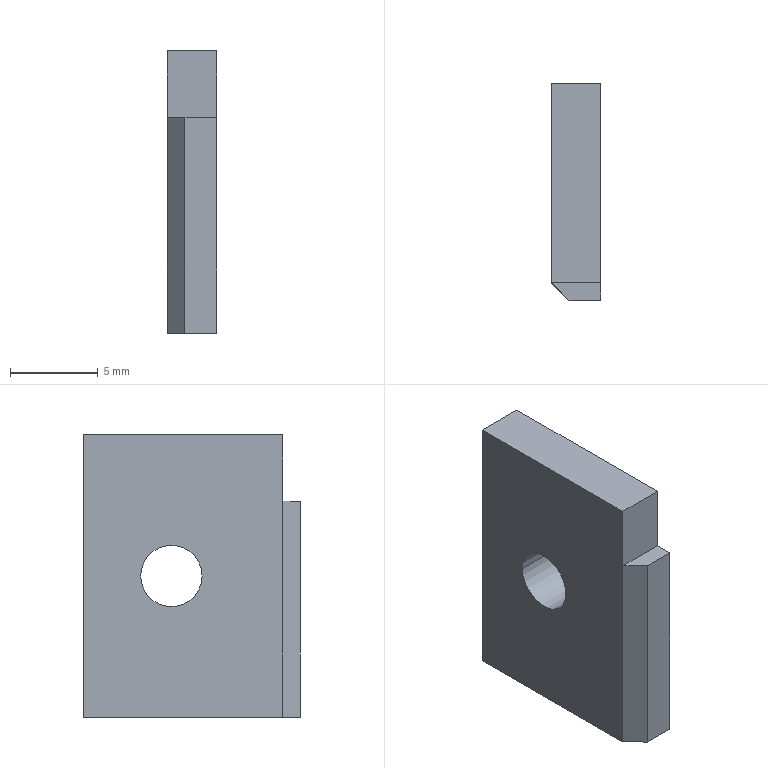Component | SolidWorks | 7.1.02.0001.00.00-0084-1 | 1 solid | 11 faces | box 2.8 x 12.35 x 16.1 mm | volume 513 mm3 | plane 9 | cylinder 2 | commonest cylinder face diameters 3.5 x2
build123d program:
from build123d import *

# Parameters (mm, degrees)
SKETCH1_W           = 12.35
SKETCH1_H           = 16.1
SKETCH1_R           = 1.75
BOSS_EXTRUDE1_DEPTH = 2.8
CHAMFER1_SIZE       = 1
SKETCH2_W           = 1
SKETCH2_H           = 3.8
CUT_EXTRUDE1_DEPTH  = 11.525


with BuildPart() as part:
    # Sketch1 → Boss-Extrude1 (new body)
    with BuildSketch(Plane.XY):
        Rectangle(SKETCH1_W, SKETCH1_H)
        with Locations((-1.175, 0)):
            Circle(SKETCH1_R, mode=Mode.SUBTRACT)
    extrude(amount=BOSS_EXTRUDE1_DEPTH)

    # Chamfer1
    chamfer1_edges = [part.edges().sort_by_distance(p)[0] for p in [
        (6.175, 0, 0),
    ]]
    chamfer(chamfer1_edges, length=CHAMFER1_SIZE)

    # Sketch2 → Cut-Extrude1 (cut, through all)
    with BuildSketch(Plane(origin=(0, 0, 0), x_dir=(-1, 0, 0), z_dir=(0, 0, -1))):
        with Locations((-5.675, -6.15)):
            Rectangle(SKETCH2_W, SKETCH2_H)
    extrude(amount=-CUT_EXTRUDE1_DEPTH, mode=Mode.SUBTRACT)


solid = part.part

# Placed as in the assembly
solid = solid.moved(Location((-67.964, 37.141, 0), (-90, 90, 0)))
STEP:
#1=COLOUR_RGB('',0.7922,0.8196,0.9333);
#2=FILL_AREA_STYLE_COLOUR('',#1);
#3=FILL_AREA_STYLE('',(#2));
#4=SURFACE_STYLE_FILL_AREA(#3);
#5=SURFACE_SIDE_STYLE('',(#4));
#6=SURFACE_STYLE_USAGE(.BOTH.,#5);
#7=PRESENTATION_STYLE_ASSIGNMENT((#6));
#8=CARTESIAN_POINT('',(-2.566,1.577,-0.));
#9=VERTEX_POINT('',#8);
#10=CARTESIAN_POINT('',(-2.566,1.44,-0.));
#11=VERTEX_POINT('',#10);
#12=CARTESIAN_POINT('',(-2.566,1.509,-0.));
#13=DIRECTION('',(1.,-0.,-0.));
#14=DIRECTION('',(0.,-1.,-0.));
#15=AXIS2_PLACEMENT_3D('',#12,#13,#14);
#16=CIRCLE('',#15,0.0689);
#17=EDGE_CURVE('',#9,#11,#16,.T.);
#18=ORIENTED_EDGE('',*,*,#17,.T.);
#19=CARTESIAN_POINT('',(-2.676,1.44,-0.));
#20=VERTEX_POINT('',#19);
#21=CARTESIAN_POINT('',(-2.566,1.44,-0.));
#22=DIRECTION('',(-1.,0.,0.));
#23=VECTOR('',#22,39.37);
#24=LINE('',#21,#23);
#25=EDGE_CURVE('',#11,#20,#24,.T.);
#26=ORIENTED_EDGE('',*,*,#25,.T.);
#27=CARTESIAN_POINT('',(-2.676,1.577,-0.));
#28=VERTEX_POINT('',#27);
#29=CARTESIAN_POINT('',(-2.676,1.509,-0.));
#30=DIRECTION('',(1.,-0.,-0.));
#31=DIRECTION('',(0.,-1.,-0.));
#32=AXIS2_PLACEMENT_3D('',#29,#30,#31);
#33=CIRCLE('',#32,0.0689);
#34=EDGE_CURVE('',#28,#20,#33,.T.);
#35=ORIENTED_EDGE('',*,*,#34,.F.);
#36=CARTESIAN_POINT('',(-2.566,1.577,-0.));
#37=DIRECTION('',(-1.,0.,0.));
#38=VECTOR('',#37,39.37);
#39=LINE('',#36,#38);
#40=EDGE_CURVE('',#9,#28,#39,.T.);
#41=ORIENTED_EDGE('',*,*,#40,.F.);
#42=EDGE_LOOP('',(#18,#26,#35,#41));
#43=FACE_OUTER_BOUND('',#42,.T.);
#44=CARTESIAN_POINT('',(-2.566,1.509,-0.));
#45=DIRECTION('',(-1.,0.,0.));
#46=DIRECTION('',(0.,1.,0.));
#47=AXIS2_PLACEMENT_3D('',#44,#45,#46);
#48=CYLINDRICAL_SURFACE('',#47,0.0689);
#49=ADVANCED_FACE('',(#43),#48,.F.);
#50=CARTESIAN_POINT('',(-2.566,1.259,0.1673));
#51=VERTEX_POINT('',#50);
#52=CARTESIAN_POINT('',(-2.566,1.219,0.1673));
#53=VERTEX_POINT('',#52);
#54=CARTESIAN_POINT('',(-2.566,1.219,0.1673));
#55=DIRECTION('',(-0.,-1.,-0.));
#56=VECTOR('',#55,39.37);
#57=LINE('',#54,#56);
#58=EDGE_CURVE('',#51,#53,#57,.T.);
#59=ORIENTED_EDGE('',*,*,#58,.T.);
#60=CARTESIAN_POINT('',(-2.566,1.219,-0.3169));
#61=VERTEX_POINT('',#60);
#62=CARTESIAN_POINT('',(-2.566,1.219,-0.3169));
#63=DIRECTION('',(-0.,0.,-1.));
#64=VECTOR('',#63,39.37);
#65=LINE('',#62,#64);
#66=EDGE_CURVE('',#53,#61,#65,.T.);
#67=ORIENTED_EDGE('',*,*,#66,.T.);
#68=CARTESIAN_POINT('',(-2.566,1.705,-0.3169));
#69=VERTEX_POINT('',#68);
#70=CARTESIAN_POINT('',(-2.566,1.705,-0.3169));
#71=DIRECTION('',(0.,1.,0.));
#72=VECTOR('',#71,39.37);
#73=LINE('',#70,#72);
#74=EDGE_CURVE('',#61,#69,#73,.T.);
#75=ORIENTED_EDGE('',*,*,#74,.T.);
#76=CARTESIAN_POINT('',(-2.566,1.705,0.3169));
#77=VERTEX_POINT('',#76);
#78=CARTESIAN_POINT('',(-2.566,1.705,-0.3169));
#79=DIRECTION('',(0.,-0.,1.));
#80=VECTOR('',#79,39.37);
#81=LINE('',#78,#80);
#82=EDGE_CURVE('',#69,#77,#81,.T.);
#83=ORIENTED_EDGE('',*,*,#82,.T.);
#84=CARTESIAN_POINT('',(-2.566,1.259,0.3169));
#85=VERTEX_POINT('',#84);
#86=CARTESIAN_POINT('',(-2.566,1.705,0.3169));
#87=DIRECTION('',(-0.,-1.,-0.));
#88=VECTOR('',#87,39.37);
#89=LINE('',#86,#88);
#90=EDGE_CURVE('',#77,#85,#89,.T.);
#91=ORIENTED_EDGE('',*,*,#90,.T.);
#92=CARTESIAN_POINT('',(-2.566,1.259,0.3169));
#93=DIRECTION('',(-0.,-0.,-1.));
#94=VECTOR('',#93,39.37);
#95=LINE('',#92,#94);
#96=EDGE_CURVE('',#85,#51,#95,.T.);
#97=ORIENTED_EDGE('',*,*,#96,.T.);
#98=EDGE_LOOP('',(#59,#67,#75,#83,#91,#97));
#99=FACE_OUTER_BOUND('',#98,.T.);
#100=ORIENTED_EDGE('',*,*,#17,.F.);
#101=CARTESIAN_POINT('',(-2.566,1.509,-0.));
#102=DIRECTION('',(1.,-0.,-0.));
#103=DIRECTION('',(0.,-1.,-0.));
#104=AXIS2_PLACEMENT_3D('',#101,#102,#103);
#105=CIRCLE('',#104,0.0689);
#106=EDGE_CURVE('',#11,#9,#105,.T.);
#107=ORIENTED_EDGE('',*,*,#106,.F.);
#108=EDGE_LOOP('',(#100,#107));
#109=FACE_BOUND('',#108,.T.);
#110=CARTESIAN_POINT('',(-2.566,1.462,-0.));
#111=DIRECTION('',(1.,-0.,-0.));
#112=DIRECTION('',(-0.,-1.,-0.));
#113=AXIS2_PLACEMENT_3D('',#110,#111,#112);
#114=PLANE('',#113);
#115=ADVANCED_FACE('',(#99,#109),#114,.T.);
#116=CARTESIAN_POINT('',(-2.676,1.259,-0.3169));
#117=VERTEX_POINT('',#116);
#118=CARTESIAN_POINT('',(-2.676,1.705,-0.3169));
#119=VERTEX_POINT('',#118);
#120=CARTESIAN_POINT('',(-2.676,1.705,-0.3169));
#121=DIRECTION('',(0.,1.,0.));
#122=VECTOR('',#121,39.37);
#123=LINE('',#120,#122);
#124=EDGE_CURVE('',#117,#119,#123,.T.);
#125=ORIENTED_EDGE('',*,*,#124,.F.);
#126=CARTESIAN_POINT('',(-2.676,1.259,0.1673));
#127=VERTEX_POINT('',#126);
#128=CARTESIAN_POINT('',(-2.676,1.259,-0.));
#129=DIRECTION('',(0.,-0.,1.));
#130=VECTOR('',#129,39.37);
#131=LINE('',#128,#130);
#132=EDGE_CURVE('',#117,#127,#131,.T.);
#133=ORIENTED_EDGE('',*,*,#132,.T.);
#134=CARTESIAN_POINT('',(-2.676,1.259,0.3169));
#135=VERTEX_POINT('',#134);
#136=CARTESIAN_POINT('',(-2.676,1.259,0.3169));
#137=DIRECTION('',(-0.,-0.,-1.));
#138=VECTOR('',#137,39.37);
#139=LINE('',#136,#138);
#140=EDGE_CURVE('',#135,#127,#139,.T.);
#141=ORIENTED_EDGE('',*,*,#140,.F.);
#142=CARTESIAN_POINT('',(-2.676,1.705,0.3169));
#143=VERTEX_POINT('',#142);
#144=CARTESIAN_POINT('',(-2.676,1.705,0.3169));
#145=DIRECTION('',(-0.,-1.,-0.));
#146=VECTOR('',#145,39.37);
#147=LINE('',#144,#146);
#148=EDGE_CURVE('',#143,#135,#147,.T.);
#149=ORIENTED_EDGE('',*,*,#148,.F.);
#150=CARTESIAN_POINT('',(-2.676,1.705,-0.3169));
#151=DIRECTION('',(0.,-0.,1.));
#152=VECTOR('',#151,39.37);
#153=LINE('',#150,#152);
#154=EDGE_CURVE('',#119,#143,#153,.T.);
#155=ORIENTED_EDGE('',*,*,#154,.F.);
#156=EDGE_LOOP('',(#125,#133,#141,#149,#155));
#157=FACE_OUTER_BOUND('',#156,.T.);
#158=ORIENTED_EDGE('',*,*,#34,.T.);
#159=CARTESIAN_POINT('',(-2.676,1.509,-0.));
#160=DIRECTION('',(1.,-0.,-0.));
#161=DIRECTION('',(0.,-1.,-0.));
#162=AXIS2_PLACEMENT_3D('',#159,#160,#161);
#163=CIRCLE('',#162,0.0689);
#164=EDGE_CURVE('',#20,#28,#163,.T.);
#165=ORIENTED_EDGE('',*,*,#164,.T.);
#166=EDGE_LOOP('',(#158,#165));
#167=FACE_BOUND('',#166,.T.);
#168=CARTESIAN_POINT('',(-2.676,1.462,-0.));
#169=DIRECTION('',(1.,-0.,-0.));
#170=DIRECTION('',(-0.,-1.,-0.));
#171=AXIS2_PLACEMENT_3D('',#168,#169,#170);
#172=PLANE('',#171);
#173=ADVANCED_FACE('',(#157,#167),#172,.F.);
#174=ORIENTED_EDGE('',*,*,#154,.T.);
#175=CARTESIAN_POINT('',(-2.566,1.705,0.3169));
#176=DIRECTION('',(-1.,0.,0.));
#177=VECTOR('',#176,39.37);
#178=LINE('',#175,#177);
#179=EDGE_CURVE('',#77,#143,#178,.T.);
#180=ORIENTED_EDGE('',*,*,#179,.F.);
#181=ORIENTED_EDGE('',*,*,#82,.F.);
#182=CARTESIAN_POINT('',(-2.566,1.705,-0.3169));
#183=DIRECTION('',(-1.,0.,0.));
#184=VECTOR('',#183,39.37);
#185=LINE('',#182,#184);
#186=EDGE_CURVE('',#69,#119,#185,.T.);
#187=ORIENTED_EDGE('',*,*,#186,.T.);
#188=EDGE_LOOP('',(#174,#180,#181,#187));
#189=FACE_OUTER_BOUND('',#188,.T.);
#190=CARTESIAN_POINT('',(-2.566,1.705,-0.3169));
#191=DIRECTION('',(-0.,-1.,-0.));
#192=DIRECTION('',(-1.,0.,0.));
#193=AXIS2_PLACEMENT_3D('',#190,#191,#192);
#194=PLANE('',#193);
#195=ADVANCED_FACE('',(#189),#194,.F.);
#196=ORIENTED_EDGE('',*,*,#148,.T.);
#197=CARTESIAN_POINT('',(-2.566,1.259,0.3169));
#198=DIRECTION('',(-1.,0.,0.));
#199=VECTOR('',#198,39.37);
#200=LINE('',#197,#199);
#201=EDGE_CURVE('',#85,#135,#200,.T.);
#202=ORIENTED_EDGE('',*,*,#201,.F.);
#203=ORIENTED_EDGE('',*,*,#90,.F.);
#204=ORIENTED_EDGE('',*,*,#179,.T.);
#205=EDGE_LOOP('',(#196,#202,#203,#204));
#206=FACE_OUTER_BOUND('',#205,.T.);
#207=CARTESIAN_POINT('',(-2.566,1.705,0.3169));
#208=DIRECTION('',(-0.,0.,-1.));
#209=DIRECTION('',(1.,-0.,-0.));
#210=AXIS2_PLACEMENT_3D('',#207,#208,#209);
#211=PLANE('',#210);
#212=ADVANCED_FACE('',(#206),#211,.F.);
#213=ORIENTED_EDGE('',*,*,#66,.F.);
#214=CARTESIAN_POINT('',(-2.636,1.219,0.1673));
#215=VERTEX_POINT('',#214);
#216=CARTESIAN_POINT('',(-2.566,1.219,0.1673));
#217=DIRECTION('',(-1.,0.,0.));
#218=VECTOR('',#217,39.37);
#219=LINE('',#216,#218);
#220=EDGE_CURVE('',#53,#215,#219,.T.);
#221=ORIENTED_EDGE('',*,*,#220,.T.);
#222=CARTESIAN_POINT('',(-2.636,1.219,-0.3169));
#223=VERTEX_POINT('',#222);
#224=CARTESIAN_POINT('',(-2.636,1.219,-0.3169));
#225=DIRECTION('',(-0.,0.,-1.));
#226=VECTOR('',#225,39.37);
#227=LINE('',#224,#226);
#228=EDGE_CURVE('',#215,#223,#227,.T.);
#229=ORIENTED_EDGE('',*,*,#228,.T.);
#230=CARTESIAN_POINT('',(-2.566,1.219,-0.3169));
#231=DIRECTION('',(-1.,0.,0.));
#232=VECTOR('',#231,39.37);
#233=LINE('',#230,#232);
#234=EDGE_CURVE('',#61,#223,#233,.T.);
#235=ORIENTED_EDGE('',*,*,#234,.F.);
#236=EDGE_LOOP('',(#213,#221,#229,#235));
#237=FACE_OUTER_BOUND('',#236,.T.);
#238=CARTESIAN_POINT('',(-2.566,1.219,-0.3169));
#239=DIRECTION('',(0.,1.,0.));
#240=DIRECTION('',(1.,-0.,-0.));
#241=AXIS2_PLACEMENT_3D('',#238,#239,#240);
#242=PLANE('',#241);
#243=ADVANCED_FACE('',(#237),#242,.F.);
#244=ORIENTED_EDGE('',*,*,#234,.T.);
#245=CARTESIAN_POINT('',(-2.636,1.219,-0.3169));
#246=DIRECTION('',(-0.7071,0.7071,0.));
#247=VECTOR('',#246,39.37);
#248=LINE('',#245,#247);
#249=EDGE_CURVE('',#223,#117,#248,.T.);
#250=ORIENTED_EDGE('',*,*,#249,.T.);
#251=ORIENTED_EDGE('',*,*,#124,.T.);
#252=ORIENTED_EDGE('',*,*,#186,.F.);
#253=ORIENTED_EDGE('',*,*,#74,.F.);
#254=EDGE_LOOP('',(#244,#250,#251,#252,#253));
#255=FACE_OUTER_BOUND('',#254,.T.);
#256=CARTESIAN_POINT('',(-2.566,1.705,-0.3169));
#257=DIRECTION('',(0.,-0.,1.));
#258=DIRECTION('',(-1.,0.,0.));
#259=AXIS2_PLACEMENT_3D('',#256,#257,#258);
#260=PLANE('',#259);
#261=ADVANCED_FACE('',(#255),#260,.F.);
#262=ORIENTED_EDGE('',*,*,#25,.F.);
#263=ORIENTED_EDGE('',*,*,#106,.T.);
#264=ORIENTED_EDGE('',*,*,#40,.T.);
#265=ORIENTED_EDGE('',*,*,#164,.F.);
#266=EDGE_LOOP('',(#262,#263,#264,#265));
#267=FACE_OUTER_BOUND('',#266,.T.);
#268=CARTESIAN_POINT('',(-2.566,1.509,-0.));
#269=DIRECTION('',(-1.,0.,0.));
#270=DIRECTION('',(0.,1.,0.));
#271=AXIS2_PLACEMENT_3D('',#268,#269,#270);
#272=CYLINDRICAL_SURFACE('',#271,0.0689);
#273=ADVANCED_FACE('',(#267),#272,.F.);
#274=CARTESIAN_POINT('',(-2.636,1.219,0.1673));
#275=DIRECTION('',(0.7071,-0.7071,-0.));
#276=VECTOR('',#275,39.37);
#277=LINE('',#274,#276);
#278=EDGE_CURVE('',#127,#215,#277,.T.);
#279=ORIENTED_EDGE('',*,*,#278,.F.);
#280=ORIENTED_EDGE('',*,*,#132,.F.);
#281=ORIENTED_EDGE('',*,*,#249,.F.);
#282=ORIENTED_EDGE('',*,*,#228,.F.);
#283=EDGE_LOOP('',(#279,#280,#281,#282));
#284=FACE_OUTER_BOUND('',#283,.T.);
#285=CARTESIAN_POINT('',(-2.636,1.219,-0.3169));
#286=DIRECTION('',(0.7071,0.7071,0.));
#287=DIRECTION('',(-0.,0.,-1.));
#288=AXIS2_PLACEMENT_3D('',#285,#286,#287);
#289=PLANE('',#288);
#290=ADVANCED_FACE('',(#284),#289,.F.);
#291=ORIENTED_EDGE('',*,*,#278,.T.);
#292=ORIENTED_EDGE('',*,*,#220,.F.);
#293=ORIENTED_EDGE('',*,*,#58,.F.);
#294=CARTESIAN_POINT('',(-2.566,1.259,0.1673));
#295=DIRECTION('',(-1.,0.,0.));
#296=VECTOR('',#295,39.37);
#297=LINE('',#294,#296);
#298=EDGE_CURVE('',#51,#127,#297,.T.);
#299=ORIENTED_EDGE('',*,*,#298,.T.);
#300=EDGE_LOOP('',(#291,#292,#293,#299));
#301=FACE_OUTER_BOUND('',#300,.T.);
#302=CARTESIAN_POINT('',(-2.566,1.219,0.1673));
#303=DIRECTION('',(-0.,0.,-1.));
#304=DIRECTION('',(1.,-0.,-0.));
#305=AXIS2_PLACEMENT_3D('',#302,#303,#304);
#306=PLANE('',#305);
#307=ADVANCED_FACE('',(#301),#306,.F.);
#308=ORIENTED_EDGE('',*,*,#140,.T.);
#309=ORIENTED_EDGE('',*,*,#298,.F.);
#310=ORIENTED_EDGE('',*,*,#96,.F.);
#311=ORIENTED_EDGE('',*,*,#201,.T.);
#312=EDGE_LOOP('',(#308,#309,#310,#311));
#313=FACE_OUTER_BOUND('',#312,.T.);
#314=CARTESIAN_POINT('',(-2.566,1.259,0.3169));
#315=DIRECTION('',(0.,1.,-0.));
#316=DIRECTION('',(0.,0.,1.));
#317=AXIS2_PLACEMENT_3D('',#314,#315,#316);
#318=PLANE('',#317);
#319=ADVANCED_FACE('',(#313),#318,.F.);
#320=CLOSED_SHELL('',(#49,#115,#173,#195,#212,#243,#261,#273,#290,#307,#319));
#321=MANIFOLD_SOLID_BREP('',#320);
#322=STYLED_ITEM('',(#7),#321);
#323=(LENGTH_UNIT()NAMED_UNIT(*)SI_UNIT($,.METRE.));
#324=LENGTH_MEASURE_WITH_UNIT(LENGTH_MEASURE(0.0254),#323);
#325=DIMENSIONAL_EXPONENTS(1.,0.,0.,0.,0.,0.,0.);
#326=(CONVERSION_BASED_UNIT('',#324)LENGTH_UNIT()NAMED_UNIT(#325));
#327=UNCERTAINTY_MEASURE_WITH_UNIT(LENGTH_MEASURE(0.00001),#326,'','');
#328=(NAMED_UNIT(*)PLANE_ANGLE_UNIT()SI_UNIT($,.RADIAN.));
#329=(NAMED_UNIT(*)SI_UNIT($,.STERADIAN.)SOLID_ANGLE_UNIT());
#330=(GEOMETRIC_REPRESENTATION_CONTEXT(3)GLOBAL_UNCERTAINTY_ASSIGNED_CONTEXT((#327))GLOBAL_UNIT_ASSIGNED_CONTEXT((#326,#328,#329))REPRESENTATION_CONTEXT('',''));
#331=MECHANICAL_DESIGN_GEOMETRIC_PRESENTATION_REPRESENTATION('',(#322),#330);
#332=PRESENTATION_LAYER_ASSIGNMENT('','',(#322));
#333=CARTESIAN_POINT('',(0.,0.,0.));
#334=DIRECTION('',(0.,0.,1.));
#335=DIRECTION('',(1.,0.,0.));
#336=AXIS2_PLACEMENT_3D('',#333,#334,#335);
#337=(LENGTH_UNIT()NAMED_UNIT(*)SI_UNIT($,.METRE.));
#338=LENGTH_MEASURE_WITH_UNIT(LENGTH_MEASURE(0.0254),#337);
#339=DIMENSIONAL_EXPONENTS(1.,0.,0.,0.,0.,0.,0.);
#340=(CONVERSION_BASED_UNIT('',#338)LENGTH_UNIT()NAMED_UNIT(#339));
#341=UNCERTAINTY_MEASURE_WITH_UNIT(LENGTH_MEASURE(0.00001),#340,'','');
#342=(NAMED_UNIT(*)PLANE_ANGLE_UNIT()SI_UNIT($,.RADIAN.));
#343=(NAMED_UNIT(*)SI_UNIT($,.STERADIAN.)SOLID_ANGLE_UNIT());
#344=(GEOMETRIC_REPRESENTATION_CONTEXT(3)GLOBAL_UNCERTAINTY_ASSIGNED_CONTEXT((#341))GLOBAL_UNIT_ASSIGNED_CONTEXT((#340,#342,#343))REPRESENTATION_CONTEXT('',''));
#345=ADVANCED_BREP_SHAPE_REPRESENTATION('',(#321,#336),#344);